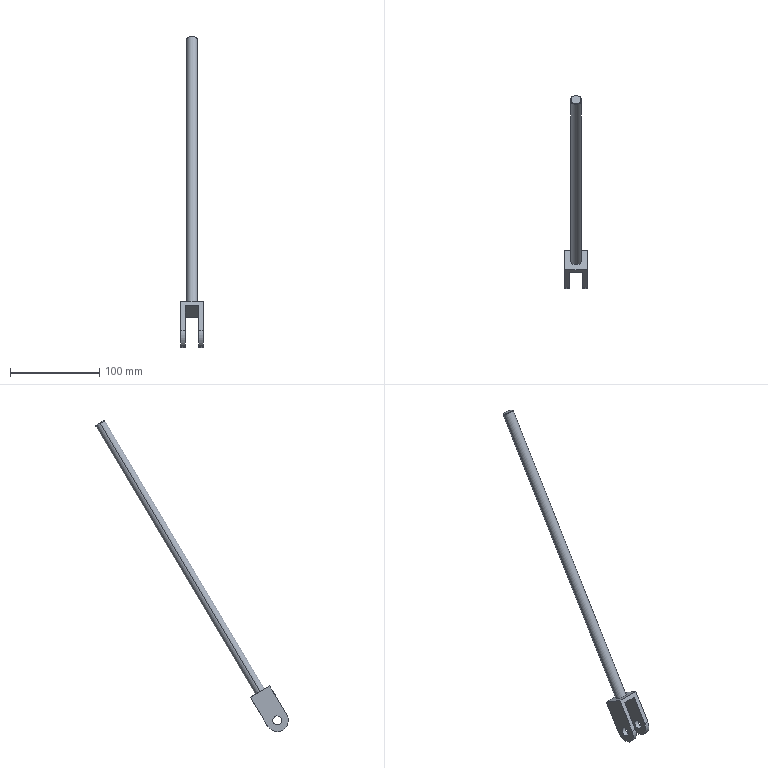Component | SolidWorks | PullRod-1 | 1 solid | 21 faces | box 25 x 215.71 x 348.22 mm | volume 52498 mm3 | cylinder 10 | plane 9 | cone 2 | commonest cylinder face diameters 10 x4 25 x4 12 x2
STEP:
#1=COLOUR_RGB('',0.7922,0.8196,0.9333);
#2=FILL_AREA_STYLE_COLOUR('',#1);
#3=FILL_AREA_STYLE('',(#2));
#4=SURFACE_STYLE_FILL_AREA(#3);
#5=SURFACE_SIDE_STYLE('',(#4));
#6=SURFACE_STYLE_USAGE(.BOTH.,#5);
#7=PRESENTATION_STYLE_ASSIGNMENT((#6));
#8=CARTESIAN_POINT('',(0.2165,5.433,2.941));
#9=VERTEX_POINT('',#8);
#10=CARTESIAN_POINT('',(-0.2165,5.433,2.941));
#11=VERTEX_POINT('',#10);
#12=CARTESIAN_POINT('',(-0.,5.433,2.941));
#13=DIRECTION('',(0.,0.5118,0.8591));
#14=DIRECTION('',(1.,0.,0.));
#15=AXIS2_PLACEMENT_3D('',#12,#13,#14);
#16=CIRCLE('',#15,0.2165);
#17=EDGE_CURVE('',#9,#11,#16,.T.);
#18=ORIENTED_EDGE('',*,*,#17,.F.);
#19=CARTESIAN_POINT('',(0.2362,5.423,2.924));
#20=VERTEX_POINT('',#19);
#21=CARTESIAN_POINT('',(0.2165,5.433,2.941));
#22=DIRECTION('',(0.7071,-0.3619,-0.6075));
#23=VECTOR('',#22,39.37);
#24=LINE('',#21,#23);
#25=EDGE_CURVE('',#9,#20,#24,.T.);
#26=ORIENTED_EDGE('',*,*,#25,.T.);
#27=CARTESIAN_POINT('',(-0.2362,5.423,2.924));
#28=VERTEX_POINT('',#27);
#29=CARTESIAN_POINT('',(-0.,5.423,2.924));
#30=DIRECTION('',(0.,-0.5118,-0.8591));
#31=DIRECTION('',(1.,0.,0.));
#32=AXIS2_PLACEMENT_3D('',#29,#30,#31);
#33=CIRCLE('',#32,0.2362);
#34=EDGE_CURVE('',#28,#20,#33,.T.);
#35=ORIENTED_EDGE('',*,*,#34,.F.);
#36=CARTESIAN_POINT('',(-0.2165,5.433,2.941));
#37=DIRECTION('',(-0.7071,-0.3619,-0.6075));
#38=VECTOR('',#37,39.37);
#39=LINE('',#36,#38);
#40=EDGE_CURVE('',#11,#28,#39,.T.);
#41=ORIENTED_EDGE('',*,*,#40,.F.);
#42=EDGE_LOOP('',(#18,#26,#35,#41));
#43=FACE_OUTER_BOUND('',#42,.T.);
#44=CARTESIAN_POINT('',(-0.,5.433,2.941));
#45=DIRECTION('',(0.,-0.5118,-0.8591));
#46=DIRECTION('',(-1.,0.,0.));
#47=AXIS2_PLACEMENT_3D('',#44,#45,#46);
#48=CONICAL_SURFACE('',#47,0.2165,0.7854);
#49=ADVANCED_FACE('',(#43),#48,.T.);
#50=CARTESIAN_POINT('',(-0.4921,-2.274,-9.997));
#51=VERTEX_POINT('',#50);
#52=CARTESIAN_POINT('',(-0.4921,-2.475,-10.335));
#53=VERTEX_POINT('',#52);
#54=CARTESIAN_POINT('',(-0.4921,-2.374,-10.166));
#55=DIRECTION('',(1.,0.,0.));
#56=DIRECTION('',(0.,-0.5118,-0.8591));
#57=AXIS2_PLACEMENT_3D('',#54,#55,#56);
#58=CIRCLE('',#57,0.1969);
#59=EDGE_CURVE('',#51,#53,#58,.T.);
#60=ORIENTED_EDGE('',*,*,#59,.F.);
#61=CARTESIAN_POINT('',(-0.2953,-2.274,-9.997));
#62=VERTEX_POINT('',#61);
#63=CARTESIAN_POINT('',(-0.4921,-2.274,-9.997));
#64=DIRECTION('',(1.,0.,0.));
#65=VECTOR('',#64,39.37);
#66=LINE('',#63,#65);
#67=EDGE_CURVE('',#51,#62,#66,.T.);
#68=ORIENTED_EDGE('',*,*,#67,.T.);
#69=CARTESIAN_POINT('',(-0.2953,-2.475,-10.335));
#70=VERTEX_POINT('',#69);
#71=CARTESIAN_POINT('',(-0.2953,-2.374,-10.166));
#72=DIRECTION('',(-1.,0.,0.));
#73=DIRECTION('',(0.,0.5118,0.8591));
#74=AXIS2_PLACEMENT_3D('',#71,#72,#73);
#75=CIRCLE('',#74,0.1969);
#76=EDGE_CURVE('',#70,#62,#75,.T.);
#77=ORIENTED_EDGE('',*,*,#76,.F.);
#78=CARTESIAN_POINT('',(-0.4921,-2.475,-10.335));
#79=DIRECTION('',(1.,0.,0.));
#80=VECTOR('',#79,39.37);
#81=LINE('',#78,#80);
#82=EDGE_CURVE('',#53,#70,#81,.T.);
#83=ORIENTED_EDGE('',*,*,#82,.F.);
#84=EDGE_LOOP('',(#60,#68,#77,#83));
#85=FACE_OUTER_BOUND('',#84,.T.);
#86=CARTESIAN_POINT('',(-0.4921,-2.374,-10.166));
#87=DIRECTION('',(1.,0.,0.));
#88=DIRECTION('',(0.,-0.5118,-0.8591));
#89=AXIS2_PLACEMENT_3D('',#86,#87,#88);
#90=CYLINDRICAL_SURFACE('',#89,0.1969);
#91=ADVANCED_FACE('',(#85),#90,.F.);
#92=CARTESIAN_POINT('',(0.2953,-2.274,-9.997));
#93=VERTEX_POINT('',#92);
#94=CARTESIAN_POINT('',(0.2953,-2.475,-10.335));
#95=VERTEX_POINT('',#94);
#96=CARTESIAN_POINT('',(0.2953,-2.374,-10.166));
#97=DIRECTION('',(1.,-0.,-0.));
#98=DIRECTION('',(0.,-0.5118,-0.8591));
#99=AXIS2_PLACEMENT_3D('',#96,#97,#98);
#100=CIRCLE('',#99,0.1969);
#101=EDGE_CURVE('',#93,#95,#100,.T.);
#102=ORIENTED_EDGE('',*,*,#101,.F.);
#103=CARTESIAN_POINT('',(0.4921,-2.274,-9.997));
#104=VERTEX_POINT('',#103);
#105=CARTESIAN_POINT('',(-0.4921,-2.274,-9.997));
#106=DIRECTION('',(1.,0.,0.));
#107=VECTOR('',#106,39.37);
#108=LINE('',#105,#107);
#109=EDGE_CURVE('',#93,#104,#108,.T.);
#110=ORIENTED_EDGE('',*,*,#109,.T.);
#111=CARTESIAN_POINT('',(0.4921,-2.475,-10.335));
#112=VERTEX_POINT('',#111);
#113=CARTESIAN_POINT('',(0.4921,-2.374,-10.166));
#114=DIRECTION('',(1.,0.,0.));
#115=DIRECTION('',(0.,-0.5118,-0.8591));
#116=AXIS2_PLACEMENT_3D('',#113,#114,#115);
#117=CIRCLE('',#116,0.1969);
#118=EDGE_CURVE('',#104,#112,#117,.T.);
#119=ORIENTED_EDGE('',*,*,#118,.T.);
#120=CARTESIAN_POINT('',(-0.4921,-2.475,-10.335));
#121=DIRECTION('',(1.,0.,0.));
#122=VECTOR('',#121,39.37);
#123=LINE('',#120,#122);
#124=EDGE_CURVE('',#95,#112,#123,.T.);
#125=ORIENTED_EDGE('',*,*,#124,.F.);
#126=EDGE_LOOP('',(#102,#110,#119,#125));
#127=FACE_OUTER_BOUND('',#126,.T.);
#128=CARTESIAN_POINT('',(-0.4921,-2.374,-10.166));
#129=DIRECTION('',(1.,0.,0.));
#130=DIRECTION('',(0.,-0.5118,-0.8591));
#131=AXIS2_PLACEMENT_3D('',#128,#129,#130);
#132=CYLINDRICAL_SURFACE('',#131,0.1969);
#133=ADVANCED_FACE('',(#127),#132,.F.);
#134=ORIENTED_EDGE('',*,*,#34,.T.);
#135=CARTESIAN_POINT('',(0.2362,-1.619,-8.898));
#136=VERTEX_POINT('',#135);
#137=CARTESIAN_POINT('',(0.2362,5.433,2.941));
#138=DIRECTION('',(0.,-0.5118,-0.8591));
#139=VECTOR('',#138,39.37);
#140=LINE('',#137,#139);
#141=EDGE_CURVE('',#20,#136,#140,.T.);
#142=ORIENTED_EDGE('',*,*,#141,.T.);
#143=CARTESIAN_POINT('',(-0.2362,-1.619,-8.898));
#144=VERTEX_POINT('',#143);
#145=CARTESIAN_POINT('',(-0.,-1.619,-8.898));
#146=DIRECTION('',(0.,-0.5118,-0.8591));
#147=DIRECTION('',(-1.,0.,0.));
#148=AXIS2_PLACEMENT_3D('',#145,#146,#147);
#149=CIRCLE('',#148,0.2362);
#150=EDGE_CURVE('',#144,#136,#149,.T.);
#151=ORIENTED_EDGE('',*,*,#150,.F.);
#152=CARTESIAN_POINT('',(-0.2362,5.433,2.941));
#153=DIRECTION('',(0.,-0.5118,-0.8591));
#154=VECTOR('',#153,39.37);
#155=LINE('',#152,#154);
#156=EDGE_CURVE('',#28,#144,#155,.T.);
#157=ORIENTED_EDGE('',*,*,#156,.F.);
#158=EDGE_LOOP('',(#134,#142,#151,#157));
#159=FACE_OUTER_BOUND('',#158,.T.);
#160=CARTESIAN_POINT('',(-0.,5.433,2.941));
#161=DIRECTION('',(0.,-0.5118,-0.8591));
#162=DIRECTION('',(-1.,0.,0.));
#163=AXIS2_PLACEMENT_3D('',#160,#161,#162);
#164=CYLINDRICAL_SURFACE('',#163,0.2362);
#165=ADVANCED_FACE('',(#159),#164,.T.);
#166=ORIENTED_EDGE('',*,*,#141,.F.);
#167=CARTESIAN_POINT('',(-0.,5.423,2.924));
#168=DIRECTION('',(0.,-0.5118,-0.8591));
#169=DIRECTION('',(1.,0.,0.));
#170=AXIS2_PLACEMENT_3D('',#167,#168,#169);
#171=CIRCLE('',#170,0.2362);
#172=EDGE_CURVE('',#20,#28,#171,.T.);
#173=ORIENTED_EDGE('',*,*,#172,.T.);
#174=ORIENTED_EDGE('',*,*,#156,.T.);
#175=CARTESIAN_POINT('',(-0.,-1.619,-8.898));
#176=DIRECTION('',(0.,-0.5118,-0.8591));
#177=DIRECTION('',(-1.,0.,0.));
#178=AXIS2_PLACEMENT_3D('',#175,#176,#177);
#179=CIRCLE('',#178,0.2362);
#180=EDGE_CURVE('',#136,#144,#179,.T.);
#181=ORIENTED_EDGE('',*,*,#180,.F.);
#182=EDGE_LOOP('',(#166,#173,#174,#181));
#183=FACE_OUTER_BOUND('',#182,.T.);
#184=CARTESIAN_POINT('',(-0.,5.433,2.941));
#185=DIRECTION('',(0.,-0.5118,-0.8591));
#186=DIRECTION('',(-1.,0.,0.));
#187=AXIS2_PLACEMENT_3D('',#184,#185,#186);
#188=CYLINDRICAL_SURFACE('',#187,0.2362);
#189=ADVANCED_FACE('',(#183),#188,.T.);
#190=CARTESIAN_POINT('',(-0.,5.433,2.941));
#191=DIRECTION('',(0.,0.5118,0.8591));
#192=DIRECTION('',(1.,0.,0.));
#193=AXIS2_PLACEMENT_3D('',#190,#191,#192);
#194=CIRCLE('',#193,0.2165);
#195=EDGE_CURVE('',#11,#9,#194,.T.);
#196=ORIENTED_EDGE('',*,*,#195,.T.);
#197=ORIENTED_EDGE('',*,*,#17,.T.);
#198=EDGE_LOOP('',(#196,#197));
#199=FACE_OUTER_BOUND('',#198,.T.);
#200=CARTESIAN_POINT('',(-0.,5.433,2.941));
#201=DIRECTION('',(0.,0.5118,0.8591));
#202=DIRECTION('',(1.,0.,0.));
#203=AXIS2_PLACEMENT_3D('',#200,#201,#202);
#204=PLANE('',#203);
#205=ADVANCED_FACE('',(#199),#204,.T.);
#206=CARTESIAN_POINT('',(-0.4921,-1.196,-9.149));
#207=VERTEX_POINT('',#206);
#208=CARTESIAN_POINT('',(-0.4921,-2.042,-8.646));
#209=VERTEX_POINT('',#208);
#210=CARTESIAN_POINT('',(-0.4921,-1.196,-9.149));
#211=DIRECTION('',(0.,-0.8591,0.5118));
#212=VECTOR('',#211,39.37);
#213=LINE('',#210,#212);
#214=EDGE_CURVE('',#207,#209,#213,.T.);
#215=ORIENTED_EDGE('',*,*,#214,.T.);
#216=CARTESIAN_POINT('',(0.4921,-2.042,-8.646));
#217=VERTEX_POINT('',#216);
#218=CARTESIAN_POINT('',(0.4921,-2.042,-8.646));
#219=DIRECTION('',(-1.,0.,0.));
#220=VECTOR('',#219,39.37);
#221=LINE('',#218,#220);
#222=EDGE_CURVE('',#217,#209,#221,.T.);
#223=ORIENTED_EDGE('',*,*,#222,.F.);
#224=CARTESIAN_POINT('',(0.4921,-1.196,-9.149));
#225=VERTEX_POINT('',#224);
#226=CARTESIAN_POINT('',(0.4921,-1.196,-9.149));
#227=DIRECTION('',(0.,-0.8591,0.5118));
#228=VECTOR('',#227,39.37);
#229=LINE('',#226,#228);
#230=EDGE_CURVE('',#225,#217,#229,.T.);
#231=ORIENTED_EDGE('',*,*,#230,.F.);
#232=CARTESIAN_POINT('',(0.4921,-1.196,-9.149));
#233=DIRECTION('',(-1.,0.,0.));
#234=VECTOR('',#233,39.37);
#235=LINE('',#232,#234);
#236=EDGE_CURVE('',#225,#207,#235,.T.);
#237=ORIENTED_EDGE('',*,*,#236,.T.);
#238=EDGE_LOOP('',(#215,#223,#231,#237));
#239=FACE_OUTER_BOUND('',#238,.T.);
#240=ORIENTED_EDGE('',*,*,#150,.T.);
#241=ORIENTED_EDGE('',*,*,#180,.T.);
#242=EDGE_LOOP('',(#240,#241));
#243=FACE_BOUND('',#242,.T.);
#244=CARTESIAN_POINT('',(0.4921,-1.196,-9.149));
#245=DIRECTION('',(0.,-0.5118,-0.8591));
#246=DIRECTION('',(-1.,0.,0.));
#247=AXIS2_PLACEMENT_3D('',#244,#245,#246);
#248=PLANE('',#247);
#249=ADVANCED_FACE('',(#239,#243),#248,.F.);
#250=CARTESIAN_POINT('',(-0.4921,-2.797,-9.914));
#251=VERTEX_POINT('',#250);
#252=CARTESIAN_POINT('',(-0.4921,-2.042,-8.646));
#253=DIRECTION('',(0.,-0.5118,-0.8591));
#254=VECTOR('',#253,39.37);
#255=LINE('',#252,#254);
#256=EDGE_CURVE('',#209,#251,#255,.T.);
#257=ORIENTED_EDGE('',*,*,#256,.T.);
#258=CARTESIAN_POINT('',(-0.2953,-2.797,-9.914));
#259=VERTEX_POINT('',#258);
#260=CARTESIAN_POINT('',(0.4921,-2.797,-9.914));
#261=DIRECTION('',(1.,0.,0.));
#262=VECTOR('',#261,39.37);
#263=LINE('',#260,#262);
#264=EDGE_CURVE('',#251,#259,#263,.T.);
#265=ORIENTED_EDGE('',*,*,#264,.T.);
#266=CARTESIAN_POINT('',(-0.2953,-2.142,-8.815));
#267=VERTEX_POINT('',#266);
#268=CARTESIAN_POINT('',(-0.2953,-2.142,-8.815));
#269=DIRECTION('',(0.,-0.5118,-0.8591));
#270=VECTOR('',#269,39.37);
#271=LINE('',#268,#270);
#272=EDGE_CURVE('',#267,#259,#271,.T.);
#273=ORIENTED_EDGE('',*,*,#272,.F.);
#274=CARTESIAN_POINT('',(0.2953,-2.142,-8.815));
#275=VERTEX_POINT('',#274);
#276=CARTESIAN_POINT('',(-0.2953,-2.142,-8.815));
#277=DIRECTION('',(-1.,0.,0.));
#278=VECTOR('',#277,39.37);
#279=LINE('',#276,#278);
#280=EDGE_CURVE('',#275,#267,#279,.T.);
#281=ORIENTED_EDGE('',*,*,#280,.F.);
#282=CARTESIAN_POINT('',(0.2953,-2.797,-9.914));
#283=VERTEX_POINT('',#282);
#284=CARTESIAN_POINT('',(0.2953,-2.142,-8.815));
#285=DIRECTION('',(0.,0.5118,0.8591));
#286=VECTOR('',#285,39.37);
#287=LINE('',#284,#286);
#288=EDGE_CURVE('',#283,#275,#287,.T.);
#289=ORIENTED_EDGE('',*,*,#288,.F.);
#290=CARTESIAN_POINT('',(0.4921,-2.797,-9.914));
#291=VERTEX_POINT('',#290);
#292=CARTESIAN_POINT('',(0.4921,-2.797,-9.914));
#293=DIRECTION('',(1.,0.,0.));
#294=VECTOR('',#293,39.37);
#295=LINE('',#292,#294);
#296=EDGE_CURVE('',#283,#291,#295,.T.);
#297=ORIENTED_EDGE('',*,*,#296,.T.);
#298=CARTESIAN_POINT('',(0.4921,-2.042,-8.646));
#299=DIRECTION('',(0.,-0.5118,-0.8591));
#300=VECTOR('',#299,39.37);
#301=LINE('',#298,#300);
#302=EDGE_CURVE('',#217,#291,#301,.T.);
#303=ORIENTED_EDGE('',*,*,#302,.F.);
#304=ORIENTED_EDGE('',*,*,#222,.T.);
#305=EDGE_LOOP('',(#257,#265,#273,#281,#289,#297,#303,#304));
#306=FACE_OUTER_BOUND('',#305,.T.);
#307=CARTESIAN_POINT('',(0.4921,-2.042,-8.646));
#308=DIRECTION('',(0.,0.8591,-0.5118));
#309=DIRECTION('',(0.,0.5118,0.8591));
#310=AXIS2_PLACEMENT_3D('',#307,#308,#309);
#311=PLANE('',#310);
#312=ADVANCED_FACE('',(#306),#311,.F.);
#313=CARTESIAN_POINT('',(0.4921,-1.952,-10.418));
#314=VERTEX_POINT('',#313);
#315=CARTESIAN_POINT('',(0.4921,-1.196,-9.149));
#316=DIRECTION('',(0.,0.5118,0.8591));
#317=VECTOR('',#316,39.37);
#318=LINE('',#315,#317);
#319=EDGE_CURVE('',#314,#225,#318,.T.);
#320=ORIENTED_EDGE('',*,*,#319,.F.);
#321=CARTESIAN_POINT('',(0.2953,-1.952,-10.418));
#322=VERTEX_POINT('',#321);
#323=CARTESIAN_POINT('',(0.4921,-1.952,-10.418));
#324=DIRECTION('',(-1.,0.,0.));
#325=VECTOR('',#324,39.37);
#326=LINE('',#323,#325);
#327=EDGE_CURVE('',#314,#322,#326,.T.);
#328=ORIENTED_EDGE('',*,*,#327,.T.);
#329=CARTESIAN_POINT('',(0.2953,-1.297,-9.319));
#330=VERTEX_POINT('',#329);
#331=CARTESIAN_POINT('',(0.2953,-1.297,-9.319));
#332=DIRECTION('',(0.,0.5118,0.8591));
#333=VECTOR('',#332,39.37);
#334=LINE('',#331,#333);
#335=EDGE_CURVE('',#322,#330,#334,.T.);
#336=ORIENTED_EDGE('',*,*,#335,.T.);
#337=CARTESIAN_POINT('',(-0.2953,-1.297,-9.319));
#338=VERTEX_POINT('',#337);
#339=CARTESIAN_POINT('',(-0.2953,-1.297,-9.319));
#340=DIRECTION('',(-1.,0.,0.));
#341=VECTOR('',#340,39.37);
#342=LINE('',#339,#341);
#343=EDGE_CURVE('',#330,#338,#342,.T.);
#344=ORIENTED_EDGE('',*,*,#343,.T.);
#345=CARTESIAN_POINT('',(-0.2953,-1.952,-10.418));
#346=VERTEX_POINT('',#345);
#347=CARTESIAN_POINT('',(-0.2953,-1.297,-9.319));
#348=DIRECTION('',(0.,-0.5118,-0.8591));
#349=VECTOR('',#348,39.37);
#350=LINE('',#347,#349);
#351=EDGE_CURVE('',#338,#346,#350,.T.);
#352=ORIENTED_EDGE('',*,*,#351,.T.);
#353=CARTESIAN_POINT('',(-0.4921,-1.952,-10.418));
#354=VERTEX_POINT('',#353);
#355=CARTESIAN_POINT('',(0.4921,-1.952,-10.418));
#356=DIRECTION('',(-1.,0.,0.));
#357=VECTOR('',#356,39.37);
#358=LINE('',#355,#357);
#359=EDGE_CURVE('',#346,#354,#358,.T.);
#360=ORIENTED_EDGE('',*,*,#359,.T.);
#361=CARTESIAN_POINT('',(-0.4921,-1.196,-9.149));
#362=DIRECTION('',(0.,0.5118,0.8591));
#363=VECTOR('',#362,39.37);
#364=LINE('',#361,#363);
#365=EDGE_CURVE('',#354,#207,#364,.T.);
#366=ORIENTED_EDGE('',*,*,#365,.T.);
#367=ORIENTED_EDGE('',*,*,#236,.F.);
#368=EDGE_LOOP('',(#320,#328,#336,#344,#352,#360,#366,#367));
#369=FACE_OUTER_BOUND('',#368,.T.);
#370=CARTESIAN_POINT('',(0.4921,-1.196,-9.149));
#371=DIRECTION('',(0.,-0.8591,0.5118));
#372=DIRECTION('',(0.,-0.5118,-0.8591));
#373=AXIS2_PLACEMENT_3D('',#370,#371,#372);
#374=PLANE('',#373);
#375=ADVANCED_FACE('',(#369),#374,.F.);
#376=CARTESIAN_POINT('',(0.4921,-2.374,-10.166));
#377=DIRECTION('',(1.,0.,0.));
#378=DIRECTION('',(0.,-0.5118,-0.8591));
#379=AXIS2_PLACEMENT_3D('',#376,#377,#378);
#380=CIRCLE('',#379,0.1969);
#381=EDGE_CURVE('',#112,#104,#380,.T.);
#382=ORIENTED_EDGE('',*,*,#381,.F.);
#383=ORIENTED_EDGE('',*,*,#118,.F.);
#384=EDGE_LOOP('',(#382,#383));
#385=FACE_BOUND('',#384,.T.);
#386=CARTESIAN_POINT('',(0.4921,-2.626,-10.589));
#387=VERTEX_POINT('',#386);
#388=CARTESIAN_POINT('',(0.4921,-2.374,-10.166));
#389=DIRECTION('',(1.,0.,0.));
#390=DIRECTION('',(0.,-0.5118,-0.8591));
#391=AXIS2_PLACEMENT_3D('',#388,#389,#390);
#392=CIRCLE('',#391,0.4921);
#393=EDGE_CURVE('',#291,#387,#392,.T.);
#394=ORIENTED_EDGE('',*,*,#393,.T.);
#395=CARTESIAN_POINT('',(0.4921,-2.374,-10.166));
#396=DIRECTION('',(1.,0.,0.));
#397=DIRECTION('',(0.,-0.5118,-0.8591));
#398=AXIS2_PLACEMENT_3D('',#395,#396,#397);
#399=CIRCLE('',#398,0.4921);
#400=EDGE_CURVE('',#387,#314,#399,.T.);
#401=ORIENTED_EDGE('',*,*,#400,.T.);
#402=ORIENTED_EDGE('',*,*,#319,.T.);
#403=ORIENTED_EDGE('',*,*,#230,.T.);
#404=ORIENTED_EDGE('',*,*,#302,.T.);
#405=EDGE_LOOP('',(#394,#401,#402,#403,#404));
#406=FACE_OUTER_BOUND('',#405,.T.);
#407=CARTESIAN_POINT('',(0.4921,1.907,-2.978));
#408=DIRECTION('',(1.,0.,0.));
#409=DIRECTION('',(0.,-0.5118,-0.8591));
#410=AXIS2_PLACEMENT_3D('',#407,#408,#409);
#411=PLANE('',#410);
#412=ADVANCED_FACE('',(#385,#406),#411,.T.);
#413=CARTESIAN_POINT('',(-0.4921,-2.374,-10.166));
#414=DIRECTION('',(1.,0.,0.));
#415=DIRECTION('',(0.,-0.5118,-0.8591));
#416=AXIS2_PLACEMENT_3D('',#413,#414,#415);
#417=CIRCLE('',#416,0.1969);
#418=EDGE_CURVE('',#53,#51,#417,.T.);
#419=ORIENTED_EDGE('',*,*,#418,.T.);
#420=ORIENTED_EDGE('',*,*,#59,.T.);
#421=EDGE_LOOP('',(#419,#420));
#422=FACE_BOUND('',#421,.T.);
#423=ORIENTED_EDGE('',*,*,#365,.F.);
#424=CARTESIAN_POINT('',(-0.4921,-2.626,-10.589));
#425=VERTEX_POINT('',#424);
#426=CARTESIAN_POINT('',(-0.4921,-2.374,-10.166));
#427=DIRECTION('',(-1.,0.,0.));
#428=DIRECTION('',(0.,-0.5118,-0.8591));
#429=AXIS2_PLACEMENT_3D('',#426,#427,#428);
#430=CIRCLE('',#429,0.4921);
#431=EDGE_CURVE('',#354,#425,#430,.T.);
#432=ORIENTED_EDGE('',*,*,#431,.T.);
#433=CARTESIAN_POINT('',(-0.4921,-2.374,-10.166));
#434=DIRECTION('',(-1.,0.,0.));
#435=DIRECTION('',(0.,-0.5118,-0.8591));
#436=AXIS2_PLACEMENT_3D('',#433,#434,#435);
#437=CIRCLE('',#436,0.4921);
#438=EDGE_CURVE('',#425,#251,#437,.T.);
#439=ORIENTED_EDGE('',*,*,#438,.T.);
#440=ORIENTED_EDGE('',*,*,#256,.F.);
#441=ORIENTED_EDGE('',*,*,#214,.F.);
#442=EDGE_LOOP('',(#423,#432,#439,#440,#441));
#443=FACE_OUTER_BOUND('',#442,.T.);
#444=CARTESIAN_POINT('',(-0.4921,1.907,-2.978));
#445=DIRECTION('',(1.,0.,0.));
#446=DIRECTION('',(0.,-0.5118,-0.8591));
#447=AXIS2_PLACEMENT_3D('',#444,#445,#446);
#448=PLANE('',#447);
#449=ADVANCED_FACE('',(#422,#443),#448,.F.);
#450=ORIENTED_EDGE('',*,*,#76,.T.);
#451=CARTESIAN_POINT('',(-0.2953,-2.374,-10.166));
#452=DIRECTION('',(-1.,0.,0.));
#453=DIRECTION('',(0.,0.5118,0.8591));
#454=AXIS2_PLACEMENT_3D('',#451,#452,#453);
#455=CIRCLE('',#454,0.1969);
#456=EDGE_CURVE('',#62,#70,#455,.T.);
#457=ORIENTED_EDGE('',*,*,#456,.T.);
#458=EDGE_LOOP('',(#450,#457));
#459=FACE_BOUND('',#458,.T.);
#460=CARTESIAN_POINT('',(-0.2953,-2.626,-10.589));
#461=VERTEX_POINT('',#460);
#462=CARTESIAN_POINT('',(-0.2953,-2.374,-10.166));
#463=DIRECTION('',(1.,0.,0.));
#464=DIRECTION('',(0.,0.5118,0.8591));
#465=AXIS2_PLACEMENT_3D('',#462,#463,#464);
#466=CIRCLE('',#465,0.4921);
#467=EDGE_CURVE('',#259,#461,#466,.T.);
#468=ORIENTED_EDGE('',*,*,#467,.T.);
#469=CARTESIAN_POINT('',(-0.2953,-2.374,-10.166));
#470=DIRECTION('',(1.,0.,0.));
#471=DIRECTION('',(0.,0.5118,0.8591));
#472=AXIS2_PLACEMENT_3D('',#469,#470,#471);
#473=CIRCLE('',#472,0.4921);
#474=EDGE_CURVE('',#461,#346,#473,.T.);
#475=ORIENTED_EDGE('',*,*,#474,.T.);
#476=ORIENTED_EDGE('',*,*,#351,.F.);
#477=CARTESIAN_POINT('',(-0.2953,-1.297,-9.319));
#478=DIRECTION('',(0.,-0.8591,0.5118));
#479=VECTOR('',#478,39.37);
#480=LINE('',#477,#479);
#481=EDGE_CURVE('',#338,#267,#480,.T.);
#482=ORIENTED_EDGE('',*,*,#481,.T.);
#483=ORIENTED_EDGE('',*,*,#272,.T.);
#484=EDGE_LOOP('',(#468,#475,#476,#482,#483));
#485=FACE_OUTER_BOUND('',#484,.T.);
#486=CARTESIAN_POINT('',(-0.2953,-1.297,-9.319));
#487=DIRECTION('',(-1.,0.,0.));
#488=DIRECTION('',(0.,0.5118,0.8591));
#489=AXIS2_PLACEMENT_3D('',#486,#487,#488);
#490=PLANE('',#489);
#491=ADVANCED_FACE('',(#459,#485),#490,.F.);
#492=ORIENTED_EDGE('',*,*,#280,.T.);
#493=ORIENTED_EDGE('',*,*,#481,.F.);
#494=ORIENTED_EDGE('',*,*,#343,.F.);
#495=CARTESIAN_POINT('',(0.2953,-1.297,-9.319));
#496=DIRECTION('',(0.,-0.8591,0.5118));
#497=VECTOR('',#496,39.37);
#498=LINE('',#495,#497);
#499=EDGE_CURVE('',#330,#275,#498,.T.);
#500=ORIENTED_EDGE('',*,*,#499,.T.);
#501=EDGE_LOOP('',(#492,#493,#494,#500));
#502=FACE_OUTER_BOUND('',#501,.T.);
#503=CARTESIAN_POINT('',(-0.2953,-1.297,-9.319));
#504=DIRECTION('',(0.,0.5118,0.8591));
#505=DIRECTION('',(1.,0.,0.));
#506=AXIS2_PLACEMENT_3D('',#503,#504,#505);
#507=PLANE('',#506);
#508=ADVANCED_FACE('',(#502),#507,.F.);
#509=CARTESIAN_POINT('',(0.2953,-2.374,-10.166));
#510=DIRECTION('',(1.,-0.,-0.));
#511=DIRECTION('',(0.,-0.5118,-0.8591));
#512=AXIS2_PLACEMENT_3D('',#509,#510,#511);
#513=CIRCLE('',#512,0.1969);
#514=EDGE_CURVE('',#95,#93,#513,.T.);
#515=ORIENTED_EDGE('',*,*,#514,.T.);
#516=ORIENTED_EDGE('',*,*,#101,.T.);
#517=EDGE_LOOP('',(#515,#516));
#518=FACE_BOUND('',#517,.T.);
#519=ORIENTED_EDGE('',*,*,#335,.F.);
#520=CARTESIAN_POINT('',(0.2953,-2.626,-10.589));
#521=VERTEX_POINT('',#520);
#522=CARTESIAN_POINT('',(0.2953,-2.374,-10.166));
#523=DIRECTION('',(-1.,0.,0.));
#524=DIRECTION('',(0.,-0.5118,-0.8591));
#525=AXIS2_PLACEMENT_3D('',#522,#523,#524);
#526=CIRCLE('',#525,0.4921);
#527=EDGE_CURVE('',#322,#521,#526,.T.);
#528=ORIENTED_EDGE('',*,*,#527,.T.);
#529=CARTESIAN_POINT('',(0.2953,-2.374,-10.166));
#530=DIRECTION('',(-1.,0.,0.));
#531=DIRECTION('',(0.,-0.5118,-0.8591));
#532=AXIS2_PLACEMENT_3D('',#529,#530,#531);
#533=CIRCLE('',#532,0.4921);
#534=EDGE_CURVE('',#521,#283,#533,.T.);
#535=ORIENTED_EDGE('',*,*,#534,.T.);
#536=ORIENTED_EDGE('',*,*,#288,.T.);
#537=ORIENTED_EDGE('',*,*,#499,.F.);
#538=EDGE_LOOP('',(#519,#528,#535,#536,#537));
#539=FACE_OUTER_BOUND('',#538,.T.);
#540=CARTESIAN_POINT('',(0.2953,-1.297,-9.319));
#541=DIRECTION('',(1.,-0.,-0.));
#542=DIRECTION('',(-0.,-0.5118,-0.8591));
#543=AXIS2_PLACEMENT_3D('',#540,#541,#542);
#544=PLANE('',#543);
#545=ADVANCED_FACE('',(#518,#539),#544,.F.);
#546=CARTESIAN_POINT('',(0.4921,-2.626,-10.589));
#547=DIRECTION('',(-1.,0.,0.));
#548=VECTOR('',#547,39.37);
#549=LINE('',#546,#548);
#550=EDGE_CURVE('',#387,#521,#549,.T.);
#551=ORIENTED_EDGE('',*,*,#550,.F.);
#552=ORIENTED_EDGE('',*,*,#393,.F.);
#553=ORIENTED_EDGE('',*,*,#296,.F.);
#554=ORIENTED_EDGE('',*,*,#534,.F.);
#555=EDGE_LOOP('',(#551,#552,#553,#554));
#556=FACE_OUTER_BOUND('',#555,.T.);
#557=CARTESIAN_POINT('',(0.4921,-2.374,-10.166));
#558=DIRECTION('',(-1.,0.,0.));
#559=DIRECTION('',(0.,0.5118,0.8591));
#560=AXIS2_PLACEMENT_3D('',#557,#558,#559);
#561=CYLINDRICAL_SURFACE('',#560,0.4921);
#562=ADVANCED_FACE('',(#556),#561,.T.);
#563=ORIENTED_EDGE('',*,*,#400,.F.);
#564=ORIENTED_EDGE('',*,*,#550,.T.);
#565=ORIENTED_EDGE('',*,*,#527,.F.);
#566=ORIENTED_EDGE('',*,*,#327,.F.);
#567=EDGE_LOOP('',(#563,#564,#565,#566));
#568=FACE_OUTER_BOUND('',#567,.T.);
#569=CARTESIAN_POINT('',(0.4921,-2.374,-10.166));
#570=DIRECTION('',(-1.,0.,0.));
#571=DIRECTION('',(0.,0.5118,0.8591));
#572=AXIS2_PLACEMENT_3D('',#569,#570,#571);
#573=CYLINDRICAL_SURFACE('',#572,0.4921);
#574=ADVANCED_FACE('',(#568),#573,.T.);
#575=CARTESIAN_POINT('',(0.4921,-2.626,-10.589));
#576=DIRECTION('',(-1.,0.,0.));
#577=VECTOR('',#576,39.37);
#578=LINE('',#575,#577);
#579=EDGE_CURVE('',#461,#425,#578,.T.);
#580=ORIENTED_EDGE('',*,*,#579,.F.);
#581=ORIENTED_EDGE('',*,*,#467,.F.);
#582=ORIENTED_EDGE('',*,*,#264,.F.);
#583=ORIENTED_EDGE('',*,*,#438,.F.);
#584=EDGE_LOOP('',(#580,#581,#582,#583));
#585=FACE_OUTER_BOUND('',#584,.T.);
#586=CARTESIAN_POINT('',(0.4921,-2.374,-10.166));
#587=DIRECTION('',(-1.,0.,0.));
#588=DIRECTION('',(0.,0.5118,0.8591));
#589=AXIS2_PLACEMENT_3D('',#586,#587,#588);
#590=CYLINDRICAL_SURFACE('',#589,0.4921);
#591=ADVANCED_FACE('',(#585),#590,.T.);
#592=ORIENTED_EDGE('',*,*,#474,.F.);
#593=ORIENTED_EDGE('',*,*,#579,.T.);
#594=ORIENTED_EDGE('',*,*,#431,.F.);
#595=ORIENTED_EDGE('',*,*,#359,.F.);
#596=EDGE_LOOP('',(#592,#593,#594,#595));
#597=FACE_OUTER_BOUND('',#596,.T.);
#598=CARTESIAN_POINT('',(0.4921,-2.374,-10.166));
#599=DIRECTION('',(-1.,0.,0.));
#600=DIRECTION('',(0.,0.5118,0.8591));
#601=AXIS2_PLACEMENT_3D('',#598,#599,#600);
#602=CYLINDRICAL_SURFACE('',#601,0.4921);
#603=ADVANCED_FACE('',(#597),#602,.T.);
#604=ORIENTED_EDGE('',*,*,#109,.F.);
#605=ORIENTED_EDGE('',*,*,#514,.F.);
#606=ORIENTED_EDGE('',*,*,#124,.T.);
#607=ORIENTED_EDGE('',*,*,#381,.T.);
#608=EDGE_LOOP('',(#604,#605,#606,#607));
#609=FACE_OUTER_BOUND('',#608,.T.);
#610=CARTESIAN_POINT('',(-0.4921,-2.374,-10.166));
#611=DIRECTION('',(1.,0.,0.));
#612=DIRECTION('',(0.,-0.5118,-0.8591));
#613=AXIS2_PLACEMENT_3D('',#610,#611,#612);
#614=CYLINDRICAL_SURFACE('',#613,0.1969);
#615=ADVANCED_FACE('',(#609),#614,.F.);
#616=ORIENTED_EDGE('',*,*,#67,.F.);
#617=ORIENTED_EDGE('',*,*,#418,.F.);
#618=ORIENTED_EDGE('',*,*,#82,.T.);
#619=ORIENTED_EDGE('',*,*,#456,.F.);
#620=EDGE_LOOP('',(#616,#617,#618,#619));
#621=FACE_OUTER_BOUND('',#620,.T.);
#622=CARTESIAN_POINT('',(-0.4921,-2.374,-10.166));
#623=DIRECTION('',(1.,0.,0.));
#624=DIRECTION('',(0.,-0.5118,-0.8591));
#625=AXIS2_PLACEMENT_3D('',#622,#623,#624);
#626=CYLINDRICAL_SURFACE('',#625,0.1969);
#627=ADVANCED_FACE('',(#621),#626,.F.);
#628=ORIENTED_EDGE('',*,*,#25,.F.);
#629=ORIENTED_EDGE('',*,*,#195,.F.);
#630=ORIENTED_EDGE('',*,*,#40,.T.);
#631=ORIENTED_EDGE('',*,*,#172,.F.);
#632=EDGE_LOOP('',(#628,#629,#630,#631));
#633=FACE_OUTER_BOUND('',#632,.T.);
#634=CARTESIAN_POINT('',(-0.,5.433,2.941));
#635=DIRECTION('',(0.,-0.5118,-0.8591));
#636=DIRECTION('',(-1.,0.,0.));
#637=AXIS2_PLACEMENT_3D('',#634,#635,#636);
#638=CONICAL_SURFACE('',#637,0.2165,0.7854);
#639=ADVANCED_FACE('',(#633),#638,.T.);
#640=CLOSED_SHELL('',(#49,#91,#133,#165,#189,#205,#249,#312,#375,#412,#449,#491,#508,#545,#562,#574,#591,#603,#615,#627,#639));
#641=MANIFOLD_SOLID_BREP('',#640);
#642=STYLED_ITEM('',(#7),#641);
#643=PRESENTATION_LAYER_ASSIGNMENT('','',(#642));
#644=(LENGTH_UNIT()NAMED_UNIT(*)SI_UNIT($,.METRE.));
#645=LENGTH_MEASURE_WITH_UNIT(LENGTH_MEASURE(0.0254),#644);
#646=DIMENSIONAL_EXPONENTS(1.,0.,0.,0.,0.,0.,0.);
#647=(CONVERSION_BASED_UNIT('',#645)LENGTH_UNIT()NAMED_UNIT(#646));
#648=UNCERTAINTY_MEASURE_WITH_UNIT(LENGTH_MEASURE(0.00001),#647,'','');
#649=(NAMED_UNIT(*)PLANE_ANGLE_UNIT()SI_UNIT($,.RADIAN.));
#650=(NAMED_UNIT(*)SI_UNIT($,.STERADIAN.)SOLID_ANGLE_UNIT());
#651=(GEOMETRIC_REPRESENTATION_CONTEXT(3)GLOBAL_UNCERTAINTY_ASSIGNED_CONTEXT((#648))GLOBAL_UNIT_ASSIGNED_CONTEXT((#647,#649,#650))REPRESENTATION_CONTEXT('',''));
#652=MECHANICAL_DESIGN_GEOMETRIC_PRESENTATION_REPRESENTATION('',(#642),#651);
#653=CARTESIAN_POINT('',(0.,0.,0.));
#654=DIRECTION('',(0.,0.,1.));
#655=DIRECTION('',(1.,0.,0.));
#656=AXIS2_PLACEMENT_3D('',#653,#654,#655);
#657=(LENGTH_UNIT()NAMED_UNIT(*)SI_UNIT($,.METRE.));
#658=LENGTH_MEASURE_WITH_UNIT(LENGTH_MEASURE(0.0254),#657);
#659=DIMENSIONAL_EXPONENTS(1.,0.,0.,0.,0.,0.,0.);
#660=(CONVERSION_BASED_UNIT('',#658)LENGTH_UNIT()NAMED_UNIT(#659));
#661=UNCERTAINTY_MEASURE_WITH_UNIT(LENGTH_MEASURE(0.00001),#660,'','');
#662=(NAMED_UNIT(*)PLANE_ANGLE_UNIT()SI_UNIT($,.RADIAN.));
#663=(NAMED_UNIT(*)SI_UNIT($,.STERADIAN.)SOLID_ANGLE_UNIT());
#664=(GEOMETRIC_REPRESENTATION_CONTEXT(3)GLOBAL_UNCERTAINTY_ASSIGNED_CONTEXT((#661))GLOBAL_UNIT_ASSIGNED_CONTEXT((#660,#662,#663))REPRESENTATION_CONTEXT('',''));
#665=ADVANCED_BREP_SHAPE_REPRESENTATION('',(#641,#656),#664);